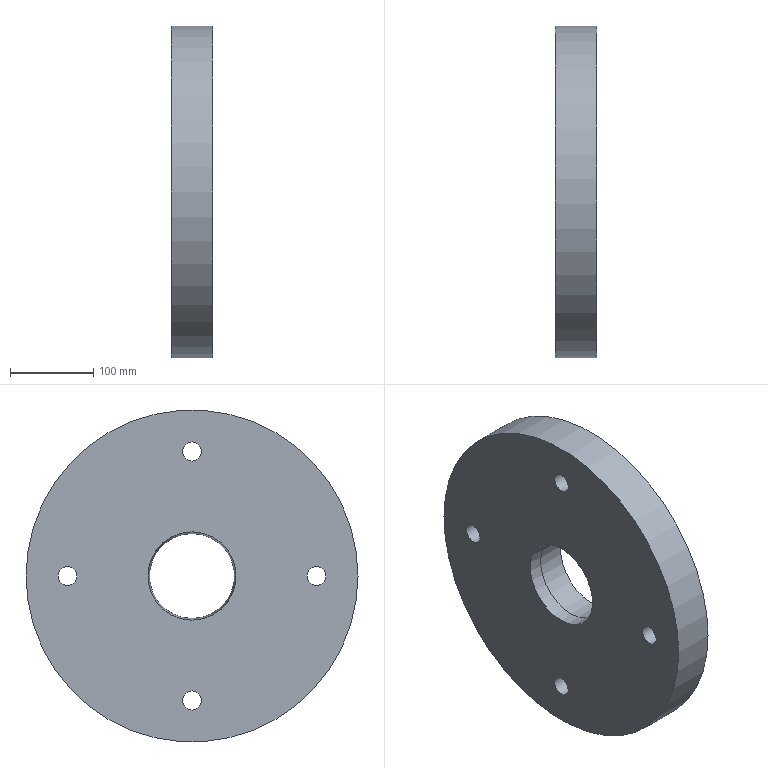Component | NX | ADAPTER_PLATE | 1 solid | 9 faces | box 50 x 400 x 400 mm | volume 5783300 mm3 | cylinder 6 | plane 2 | cone 1 | commonest cylinder face diameters 23 x4 400 x1 102.376 x1
STEP:
#1=CARTESIAN_POINT('',(0.,0.,0.));
#2=DIRECTION('',(0.,0.,1.));
#3=DIRECTION('',(1.,0.,0.));
#4=AXIS2_PLACEMENT_3D('',#1,#2,#3);
#5=CARTESIAN_POINT('',(0.,200.,-0.));
#6=VERTEX_POINT('',#5);
#7=CARTESIAN_POINT('',(0.,0.,0.));
#8=DIRECTION('',(1.,0.,0.));
#9=DIRECTION('',(0.,1.,-0.));
#10=AXIS2_PLACEMENT_3D('',#7,#8,#9);
#11=CIRCLE('',#10,200.);
#12=CARTESIAN_POINT('',(0.,0.,0.));
#13=DIRECTION('',(-1.,0.,0.));
#14=DIRECTION('',(0.,0.,1.));
#15=AXIS2_PLACEMENT_3D('',#12,#13,#14);
#16=CYLINDRICAL_SURFACE('',#15,200.);
#17=CARTESIAN_POINT('',(7.854,0.));
#18=DIRECTION('',(-1.,0.));
#19=VECTOR('',#18,1.);
#20=LINE('',#17,#19);
#21=(GEOMETRIC_REPRESENTATION_CONTEXT(2)PARAMETRIC_REPRESENTATION_CONTEXT()REPRESENTATION_CONTEXT('',''));
#22=DEFINITIONAL_REPRESENTATION('',(#20),#21);
#23=PCURVE('',#16,#22);
#24=CARTESIAN_POINT('',(0.,0.,0.));
#25=DIRECTION('',(1.,0.,0.));
#26=DIRECTION('',(0.,0.,-1.));
#27=AXIS2_PLACEMENT_3D('',#24,#25,#26);
#28=PLANE('',#27);
#29=CARTESIAN_POINT('',(0.,0.));
#30=DIRECTION('',(0.,1.));
#31=AXIS2_PLACEMENT_2D('',#29,#30);
#32=CIRCLE('',#31,200.);
#33=(GEOMETRIC_REPRESENTATION_CONTEXT(2)PARAMETRIC_REPRESENTATION_CONTEXT()REPRESENTATION_CONTEXT('',''));
#34=DEFINITIONAL_REPRESENTATION('',(#32),#33);
#35=PCURVE('',#28,#34);
#36=SURFACE_CURVE('',#11,(#23,#35),.PCURVE_S1.);
#37=EDGE_CURVE('',#6,#6,#36,.T.);
#38=ORIENTED_EDGE('',*,*,#37,.F.);
#39=CARTESIAN_POINT('',(-50.,200.,-0.));
#40=VERTEX_POINT('',#39);
#41=CARTESIAN_POINT('',(0.,200.,0.));
#42=CARTESIAN_POINT('',(-50.,200.,0.));
#43=B_SPLINE_CURVE_WITH_KNOTS('',1,(#41,#42),.UNSPECIFIED.,.F.,.F.,(2,2),(0.,50.),.PIECEWISE_BEZIER_KNOTS.);
#44=CARTESIAN_POINT('',(7.854,0.));
#45=DIRECTION('',(0.,1.));
#46=VECTOR('',#45,1.);
#47=LINE('',#44,#46);
#48=(GEOMETRIC_REPRESENTATION_CONTEXT(2)PARAMETRIC_REPRESENTATION_CONTEXT()REPRESENTATION_CONTEXT('',''));
#49=DEFINITIONAL_REPRESENTATION('',(#47),#48);
#50=PCURVE('',#16,#49);
#51=CARTESIAN_POINT('',(1.571,0.));
#52=DIRECTION('',(0.,1.));
#53=VECTOR('',#52,1.);
#54=LINE('',#51,#53);
#55=(GEOMETRIC_REPRESENTATION_CONTEXT(2)PARAMETRIC_REPRESENTATION_CONTEXT()REPRESENTATION_CONTEXT('',''));
#56=DEFINITIONAL_REPRESENTATION('',(#54),#55);
#57=PCURVE('',#16,#56);
#58=SEAM_CURVE('',#43,(#50,#57),.PCURVE_S1.);
#59=EDGE_CURVE('',#6,#40,#58,.T.);
#60=ORIENTED_EDGE('',*,*,#59,.T.);
#61=CARTESIAN_POINT('',(-50.,0.,0.));
#62=DIRECTION('',(1.,0.,0.));
#63=DIRECTION('',(0.,1.,-0.));
#64=AXIS2_PLACEMENT_3D('',#61,#62,#63);
#65=CIRCLE('',#64,200.);
#66=CARTESIAN_POINT('',(7.854,50.));
#67=DIRECTION('',(-1.,0.));
#68=VECTOR('',#67,1.);
#69=LINE('',#66,#68);
#70=(GEOMETRIC_REPRESENTATION_CONTEXT(2)PARAMETRIC_REPRESENTATION_CONTEXT()REPRESENTATION_CONTEXT('',''));
#71=DEFINITIONAL_REPRESENTATION('',(#69),#70);
#72=PCURVE('',#16,#71);
#73=CARTESIAN_POINT('',(-50.,0.,0.));
#74=DIRECTION('',(1.,0.,0.));
#75=DIRECTION('',(0.,0.,-1.));
#76=AXIS2_PLACEMENT_3D('',#73,#74,#75);
#77=PLANE('',#76);
#78=CARTESIAN_POINT('',(0.,0.));
#79=DIRECTION('',(0.,1.));
#80=AXIS2_PLACEMENT_2D('',#78,#79);
#81=CIRCLE('',#80,200.);
#82=(GEOMETRIC_REPRESENTATION_CONTEXT(2)PARAMETRIC_REPRESENTATION_CONTEXT()REPRESENTATION_CONTEXT('',''));
#83=DEFINITIONAL_REPRESENTATION('',(#81),#82);
#84=PCURVE('',#77,#83);
#85=SURFACE_CURVE('',#65,(#72,#84),.PCURVE_S1.);
#86=EDGE_CURVE('',#40,#40,#85,.T.);
#87=ORIENTED_EDGE('',*,*,#86,.T.);
#88=ORIENTED_EDGE('',*,*,#59,.F.);
#89=EDGE_LOOP('',(#38,#60,#87,#88));
#90=FACE_BOUND('',#89,.T.);
#91=ADVANCED_FACE('',(#90),#16,.T.);
#92=CARTESIAN_POINT('',(0.,150.,-11.5));
#93=VERTEX_POINT('',#92);
#94=CARTESIAN_POINT('',(0.,150.,0.));
#95=DIRECTION('',(1.,0.,0.));
#96=DIRECTION('',(0.,0.,-1.));
#97=AXIS2_PLACEMENT_3D('',#94,#95,#96);
#98=CIRCLE('',#97,11.5);
#99=CARTESIAN_POINT('',(0.,150.));
#100=DIRECTION('',(1.,0.));
#101=AXIS2_PLACEMENT_2D('',#99,#100);
#102=CIRCLE('',#101,11.5);
#103=(GEOMETRIC_REPRESENTATION_CONTEXT(2)PARAMETRIC_REPRESENTATION_CONTEXT()REPRESENTATION_CONTEXT('',''));
#104=DEFINITIONAL_REPRESENTATION('',(#102),#103);
#105=PCURVE('',#28,#104);
#106=CARTESIAN_POINT('',(-50.,150.,0.));
#107=DIRECTION('',(1.,0.,0.));
#108=DIRECTION('',(0.,0.,-1.));
#109=AXIS2_PLACEMENT_3D('',#106,#107,#108);
#110=CYLINDRICAL_SURFACE('',#109,11.5);
#111=CARTESIAN_POINT('',(0.,50.));
#112=DIRECTION('',(1.,0.));
#113=VECTOR('',#112,1.);
#114=LINE('',#111,#113);
#115=(GEOMETRIC_REPRESENTATION_CONTEXT(2)PARAMETRIC_REPRESENTATION_CONTEXT()REPRESENTATION_CONTEXT('',''));
#116=DEFINITIONAL_REPRESENTATION('',(#114),#115);
#117=PCURVE('',#110,#116);
#118=SURFACE_CURVE('',#98,(#105,#117),.PCURVE_S1.);
#119=EDGE_CURVE('',#93,#93,#118,.T.);
#120=ORIENTED_EDGE('',*,*,#119,.F.);
#121=EDGE_LOOP('',(#120));
#122=FACE_BOUND('',#121,.T.);
#123=CARTESIAN_POINT('',(0.,0.,138.5));
#124=VERTEX_POINT('',#123);
#125=CARTESIAN_POINT('',(0.,0.,150.));
#126=DIRECTION('',(1.,0.,0.));
#127=DIRECTION('',(0.,0.,-1.));
#128=AXIS2_PLACEMENT_3D('',#125,#126,#127);
#129=CIRCLE('',#128,11.5);
#130=CARTESIAN_POINT('',(-150.,0.));
#131=DIRECTION('',(1.,0.));
#132=AXIS2_PLACEMENT_2D('',#130,#131);
#133=CIRCLE('',#132,11.5);
#134=(GEOMETRIC_REPRESENTATION_CONTEXT(2)PARAMETRIC_REPRESENTATION_CONTEXT()REPRESENTATION_CONTEXT('',''));
#135=DEFINITIONAL_REPRESENTATION('',(#133),#134);
#136=PCURVE('',#28,#135);
#137=CARTESIAN_POINT('',(-50.,0.,150.));
#138=DIRECTION('',(1.,0.,0.));
#139=DIRECTION('',(0.,0.,-1.));
#140=AXIS2_PLACEMENT_3D('',#137,#138,#139);
#141=CYLINDRICAL_SURFACE('',#140,11.5);
#142=CARTESIAN_POINT('',(0.,50.));
#143=DIRECTION('',(1.,0.));
#144=VECTOR('',#143,1.);
#145=LINE('',#142,#144);
#146=(GEOMETRIC_REPRESENTATION_CONTEXT(2)PARAMETRIC_REPRESENTATION_CONTEXT()REPRESENTATION_CONTEXT('',''));
#147=DEFINITIONAL_REPRESENTATION('',(#145),#146);
#148=PCURVE('',#141,#147);
#149=SURFACE_CURVE('',#129,(#136,#148),.PCURVE_S1.);
#150=EDGE_CURVE('',#124,#124,#149,.T.);
#151=ORIENTED_EDGE('',*,*,#150,.F.);
#152=EDGE_LOOP('',(#151));
#153=FACE_BOUND('',#152,.T.);
#154=CARTESIAN_POINT('',(0.,0.,-161.5));
#155=VERTEX_POINT('',#154);
#156=CARTESIAN_POINT('',(0.,0.,-150.));
#157=DIRECTION('',(1.,0.,0.));
#158=DIRECTION('',(0.,0.,-1.));
#159=AXIS2_PLACEMENT_3D('',#156,#157,#158);
#160=CIRCLE('',#159,11.5);
#161=CARTESIAN_POINT('',(150.,0.));
#162=DIRECTION('',(1.,0.));
#163=AXIS2_PLACEMENT_2D('',#161,#162);
#164=CIRCLE('',#163,11.5);
#165=(GEOMETRIC_REPRESENTATION_CONTEXT(2)PARAMETRIC_REPRESENTATION_CONTEXT()REPRESENTATION_CONTEXT('',''));
#166=DEFINITIONAL_REPRESENTATION('',(#164),#165);
#167=PCURVE('',#28,#166);
#168=CARTESIAN_POINT('',(-50.,0.,-150.));
#169=DIRECTION('',(1.,0.,0.));
#170=DIRECTION('',(0.,0.,-1.));
#171=AXIS2_PLACEMENT_3D('',#168,#169,#170);
#172=CYLINDRICAL_SURFACE('',#171,11.5);
#173=CARTESIAN_POINT('',(0.,50.));
#174=DIRECTION('',(1.,0.));
#175=VECTOR('',#174,1.);
#176=LINE('',#173,#175);
#177=(GEOMETRIC_REPRESENTATION_CONTEXT(2)PARAMETRIC_REPRESENTATION_CONTEXT()REPRESENTATION_CONTEXT('',''));
#178=DEFINITIONAL_REPRESENTATION('',(#176),#177);
#179=PCURVE('',#172,#178);
#180=SURFACE_CURVE('',#160,(#167,#179),.PCURVE_S1.);
#181=EDGE_CURVE('',#155,#155,#180,.T.);
#182=ORIENTED_EDGE('',*,*,#181,.F.);
#183=EDGE_LOOP('',(#182));
#184=FACE_BOUND('',#183,.T.);
#185=CARTESIAN_POINT('',(0.,-150.,-11.5));
#186=VERTEX_POINT('',#185);
#187=CARTESIAN_POINT('',(0.,-150.,0.));
#188=DIRECTION('',(1.,0.,0.));
#189=DIRECTION('',(0.,0.,-1.));
#190=AXIS2_PLACEMENT_3D('',#187,#188,#189);
#191=CIRCLE('',#190,11.5);
#192=CARTESIAN_POINT('',(0.,-150.));
#193=DIRECTION('',(1.,0.));
#194=AXIS2_PLACEMENT_2D('',#192,#193);
#195=CIRCLE('',#194,11.5);
#196=(GEOMETRIC_REPRESENTATION_CONTEXT(2)PARAMETRIC_REPRESENTATION_CONTEXT()REPRESENTATION_CONTEXT('',''));
#197=DEFINITIONAL_REPRESENTATION('',(#195),#196);
#198=PCURVE('',#28,#197);
#199=CARTESIAN_POINT('',(-50.,-150.,0.));
#200=DIRECTION('',(1.,0.,0.));
#201=DIRECTION('',(0.,0.,-1.));
#202=AXIS2_PLACEMENT_3D('',#199,#200,#201);
#203=CYLINDRICAL_SURFACE('',#202,11.5);
#204=CARTESIAN_POINT('',(0.,50.));
#205=DIRECTION('',(1.,0.));
#206=VECTOR('',#205,1.);
#207=LINE('',#204,#206);
#208=(GEOMETRIC_REPRESENTATION_CONTEXT(2)PARAMETRIC_REPRESENTATION_CONTEXT()REPRESENTATION_CONTEXT('',''));
#209=DEFINITIONAL_REPRESENTATION('',(#207),#208);
#210=PCURVE('',#203,#209);
#211=SURFACE_CURVE('',#191,(#198,#210),.PCURVE_S1.);
#212=EDGE_CURVE('',#186,#186,#211,.T.);
#213=ORIENTED_EDGE('',*,*,#212,.F.);
#214=EDGE_LOOP('',(#213));
#215=FACE_BOUND('',#214,.T.);
#216=CARTESIAN_POINT('',(0.,0.,-51.188));
#217=VERTEX_POINT('',#216);
#218=CARTESIAN_POINT('',(0.,-0.,51.188));
#219=VERTEX_POINT('',#218);
#220=CARTESIAN_POINT('',(0.,0.,0.));
#221=DIRECTION('',(-1.,0.,0.));
#222=DIRECTION('',(0.,0.,-1.));
#223=AXIS2_PLACEMENT_3D('',#220,#221,#222);
#224=CIRCLE('',#223,51.188);
#225=CARTESIAN_POINT('',(51.188,0.));
#226=CARTESIAN_POINT('',(51.188,-88.66));
#227=CARTESIAN_POINT('',(-25.594,-44.33));
#228=CARTESIAN_POINT('',(-102.376,-0.));
#229=CARTESIAN_POINT('',(-25.594,44.33));
#230=CARTESIAN_POINT('',(51.188,88.66));
#231=CARTESIAN_POINT('',(51.188,0.));
#232=(BOUNDED_CURVE()B_SPLINE_CURVE(2,(#225,#226,#227,#228,#229,#230,#231),.UNSPECIFIED.,.T.,.F.)B_SPLINE_CURVE_WITH_KNOTS((1,2,2,2,2,1),(-2.094,0.,2.094,4.189,6.283,8.378),.UNSPECIFIED.)CURVE()GEOMETRIC_REPRESENTATION_ITEM()RATIONAL_B_SPLINE_CURVE((1.,0.5,1.,0.5,1.,0.5,1.))REPRESENTATION_ITEM(''));
#233=(GEOMETRIC_REPRESENTATION_CONTEXT(2)PARAMETRIC_REPRESENTATION_CONTEXT()REPRESENTATION_CONTEXT('',''));
#234=DEFINITIONAL_REPRESENTATION('',(#232),#233);
#235=PCURVE('',#28,#234);
#236=CARTESIAN_POINT('',(0.,0.,0.));
#237=DIRECTION('',(-1.,0.,0.));
#238=DIRECTION('',(0.,0.,1.));
#239=AXIS2_PLACEMENT_3D('',#236,#237,#238);
#240=CYLINDRICAL_SURFACE('',#239,51.188);
#241=CARTESIAN_POINT('',(3.142,0.));
#242=DIRECTION('',(1.,0.));
#243=VECTOR('',#242,1.);
#244=LINE('',#241,#243);
#245=(GEOMETRIC_REPRESENTATION_CONTEXT(2)PARAMETRIC_REPRESENTATION_CONTEXT()REPRESENTATION_CONTEXT('',''));
#246=DEFINITIONAL_REPRESENTATION('',(#244),#245);
#247=PCURVE('',#240,#246);
#248=SURFACE_CURVE('',#224,(#235,#247),.PCURVE_S1.);
#249=EDGE_CURVE('',#217,#219,#248,.T.);
#250=ORIENTED_EDGE('',*,*,#249,.T.);
#251=CARTESIAN_POINT('',(0.,0.,0.));
#252=DIRECTION('',(-1.,0.,0.));
#253=DIRECTION('',(0.,0.,-1.));
#254=AXIS2_PLACEMENT_3D('',#251,#252,#253);
#255=CIRCLE('',#254,51.188);
#256=CARTESIAN_POINT('',(51.188,0.));
#257=CARTESIAN_POINT('',(51.188,-88.66));
#258=CARTESIAN_POINT('',(-25.594,-44.33));
#259=CARTESIAN_POINT('',(-102.376,-0.));
#260=CARTESIAN_POINT('',(-25.594,44.33));
#261=CARTESIAN_POINT('',(51.188,88.66));
#262=CARTESIAN_POINT('',(51.188,0.));
#263=(BOUNDED_CURVE()B_SPLINE_CURVE(2,(#256,#257,#258,#259,#260,#261,#262),.UNSPECIFIED.,.T.,.F.)B_SPLINE_CURVE_WITH_KNOTS((1,2,2,2,2,1),(-2.094,0.,2.094,4.189,6.283,8.378),.UNSPECIFIED.)CURVE()GEOMETRIC_REPRESENTATION_ITEM()RATIONAL_B_SPLINE_CURVE((1.,0.5,1.,0.5,1.,0.5,1.))REPRESENTATION_ITEM(''));
#264=(GEOMETRIC_REPRESENTATION_CONTEXT(2)PARAMETRIC_REPRESENTATION_CONTEXT()REPRESENTATION_CONTEXT('',''));
#265=DEFINITIONAL_REPRESENTATION('',(#263),#264);
#266=PCURVE('',#28,#265);
#267=CARTESIAN_POINT('',(-3.142,0.));
#268=DIRECTION('',(1.,0.));
#269=VECTOR('',#268,1.);
#270=LINE('',#267,#269);
#271=(GEOMETRIC_REPRESENTATION_CONTEXT(2)PARAMETRIC_REPRESENTATION_CONTEXT()REPRESENTATION_CONTEXT('',''));
#272=DEFINITIONAL_REPRESENTATION('',(#270),#271);
#273=PCURVE('',#240,#272);
#274=SURFACE_CURVE('',#255,(#266,#273),.PCURVE_S1.);
#275=EDGE_CURVE('',#219,#217,#274,.T.);
#276=ORIENTED_EDGE('',*,*,#275,.T.);
#277=EDGE_LOOP('',(#250,#276));
#278=FACE_BOUND('',#277,.T.);
#279=ORIENTED_EDGE('',*,*,#37,.T.);
#280=EDGE_LOOP('',(#279));
#281=FACE_BOUND('',#280,.T.);
#282=ADVANCED_FACE('',(#122,#153,#184,#215,#278,#281),#28,.T.);
#283=CARTESIAN_POINT('',(-50.,150.,-11.5));
#284=VERTEX_POINT('',#283);
#285=CARTESIAN_POINT('',(-50.,150.,0.));
#286=DIRECTION('',(1.,0.,0.));
#287=DIRECTION('',(0.,0.,-1.));
#288=AXIS2_PLACEMENT_3D('',#285,#286,#287);
#289=CIRCLE('',#288,11.5);
#290=CARTESIAN_POINT('',(0.,150.));
#291=DIRECTION('',(1.,0.));
#292=AXIS2_PLACEMENT_2D('',#290,#291);
#293=CIRCLE('',#292,11.5);
#294=(GEOMETRIC_REPRESENTATION_CONTEXT(2)PARAMETRIC_REPRESENTATION_CONTEXT()REPRESENTATION_CONTEXT('',''));
#295=DEFINITIONAL_REPRESENTATION('',(#293),#294);
#296=PCURVE('',#77,#295);
#297=CARTESIAN_POINT('',(0.,0.));
#298=DIRECTION('',(1.,0.));
#299=VECTOR('',#298,1.);
#300=LINE('',#297,#299);
#301=(GEOMETRIC_REPRESENTATION_CONTEXT(2)PARAMETRIC_REPRESENTATION_CONTEXT()REPRESENTATION_CONTEXT('',''));
#302=DEFINITIONAL_REPRESENTATION('',(#300),#301);
#303=PCURVE('',#110,#302);
#304=SURFACE_CURVE('',#289,(#296,#303),.PCURVE_S1.);
#305=EDGE_CURVE('',#284,#284,#304,.T.);
#306=ORIENTED_EDGE('',*,*,#305,.T.);
#307=EDGE_LOOP('',(#306));
#308=FACE_BOUND('',#307,.T.);
#309=CARTESIAN_POINT('',(-50.,0.,138.5));
#310=VERTEX_POINT('',#309);
#311=CARTESIAN_POINT('',(-50.,0.,150.));
#312=DIRECTION('',(1.,0.,0.));
#313=DIRECTION('',(0.,0.,-1.));
#314=AXIS2_PLACEMENT_3D('',#311,#312,#313);
#315=CIRCLE('',#314,11.5);
#316=CARTESIAN_POINT('',(-150.,0.));
#317=DIRECTION('',(1.,0.));
#318=AXIS2_PLACEMENT_2D('',#316,#317);
#319=CIRCLE('',#318,11.5);
#320=(GEOMETRIC_REPRESENTATION_CONTEXT(2)PARAMETRIC_REPRESENTATION_CONTEXT()REPRESENTATION_CONTEXT('',''));
#321=DEFINITIONAL_REPRESENTATION('',(#319),#320);
#322=PCURVE('',#77,#321);
#323=CARTESIAN_POINT('',(0.,0.));
#324=DIRECTION('',(1.,0.));
#325=VECTOR('',#324,1.);
#326=LINE('',#323,#325);
#327=(GEOMETRIC_REPRESENTATION_CONTEXT(2)PARAMETRIC_REPRESENTATION_CONTEXT()REPRESENTATION_CONTEXT('',''));
#328=DEFINITIONAL_REPRESENTATION('',(#326),#327);
#329=PCURVE('',#141,#328);
#330=SURFACE_CURVE('',#315,(#322,#329),.PCURVE_S1.);
#331=EDGE_CURVE('',#310,#310,#330,.T.);
#332=ORIENTED_EDGE('',*,*,#331,.T.);
#333=EDGE_LOOP('',(#332));
#334=FACE_BOUND('',#333,.T.);
#335=CARTESIAN_POINT('',(-50.,0.,-161.5));
#336=VERTEX_POINT('',#335);
#337=CARTESIAN_POINT('',(-50.,0.,-150.));
#338=DIRECTION('',(1.,0.,0.));
#339=DIRECTION('',(0.,0.,-1.));
#340=AXIS2_PLACEMENT_3D('',#337,#338,#339);
#341=CIRCLE('',#340,11.5);
#342=CARTESIAN_POINT('',(150.,0.));
#343=DIRECTION('',(1.,0.));
#344=AXIS2_PLACEMENT_2D('',#342,#343);
#345=CIRCLE('',#344,11.5);
#346=(GEOMETRIC_REPRESENTATION_CONTEXT(2)PARAMETRIC_REPRESENTATION_CONTEXT()REPRESENTATION_CONTEXT('',''));
#347=DEFINITIONAL_REPRESENTATION('',(#345),#346);
#348=PCURVE('',#77,#347);
#349=CARTESIAN_POINT('',(0.,0.));
#350=DIRECTION('',(1.,0.));
#351=VECTOR('',#350,1.);
#352=LINE('',#349,#351);
#353=(GEOMETRIC_REPRESENTATION_CONTEXT(2)PARAMETRIC_REPRESENTATION_CONTEXT()REPRESENTATION_CONTEXT('',''));
#354=DEFINITIONAL_REPRESENTATION('',(#352),#353);
#355=PCURVE('',#172,#354);
#356=SURFACE_CURVE('',#341,(#348,#355),.PCURVE_S1.);
#357=EDGE_CURVE('',#336,#336,#356,.T.);
#358=ORIENTED_EDGE('',*,*,#357,.T.);
#359=EDGE_LOOP('',(#358));
#360=FACE_BOUND('',#359,.T.);
#361=CARTESIAN_POINT('',(-50.,-150.,-11.5));
#362=VERTEX_POINT('',#361);
#363=CARTESIAN_POINT('',(-50.,-150.,0.));
#364=DIRECTION('',(1.,0.,0.));
#365=DIRECTION('',(0.,0.,-1.));
#366=AXIS2_PLACEMENT_3D('',#363,#364,#365);
#367=CIRCLE('',#366,11.5);
#368=CARTESIAN_POINT('',(0.,-150.));
#369=DIRECTION('',(1.,0.));
#370=AXIS2_PLACEMENT_2D('',#368,#369);
#371=CIRCLE('',#370,11.5);
#372=(GEOMETRIC_REPRESENTATION_CONTEXT(2)PARAMETRIC_REPRESENTATION_CONTEXT()REPRESENTATION_CONTEXT('',''));
#373=DEFINITIONAL_REPRESENTATION('',(#371),#372);
#374=PCURVE('',#77,#373);
#375=CARTESIAN_POINT('',(0.,0.));
#376=DIRECTION('',(1.,0.));
#377=VECTOR('',#376,1.);
#378=LINE('',#375,#377);
#379=(GEOMETRIC_REPRESENTATION_CONTEXT(2)PARAMETRIC_REPRESENTATION_CONTEXT()REPRESENTATION_CONTEXT('',''));
#380=DEFINITIONAL_REPRESENTATION('',(#378),#379);
#381=PCURVE('',#203,#380);
#382=SURFACE_CURVE('',#367,(#374,#381),.PCURVE_S1.);
#383=EDGE_CURVE('',#362,#362,#382,.T.);
#384=ORIENTED_EDGE('',*,*,#383,.T.);
#385=EDGE_LOOP('',(#384));
#386=FACE_BOUND('',#385,.T.);
#387=CARTESIAN_POINT('',(-50.,0.,53.187));
#388=VERTEX_POINT('',#387);
#389=CARTESIAN_POINT('',(-50.,0.,0.));
#390=DIRECTION('',(-1.,0.,0.));
#391=DIRECTION('',(0.,0.,1.));
#392=AXIS2_PLACEMENT_3D('',#389,#390,#391);
#393=CIRCLE('',#392,53.187);
#394=CARTESIAN_POINT('',(-53.187,0.));
#395=CARTESIAN_POINT('',(-53.187,92.122));
#396=CARTESIAN_POINT('',(26.593,46.061));
#397=CARTESIAN_POINT('',(106.373,0.));
#398=CARTESIAN_POINT('',(26.593,-46.061));
#399=CARTESIAN_POINT('',(-53.187,-92.122));
#400=CARTESIAN_POINT('',(-53.187,0.));
#401=(BOUNDED_CURVE()B_SPLINE_CURVE(2,(#394,#395,#396,#397,#398,#399,#400),.UNSPECIFIED.,.T.,.F.)B_SPLINE_CURVE_WITH_KNOTS((1,2,2,2,2,1),(-2.094,0.,2.094,4.189,6.283,8.378),.UNSPECIFIED.)CURVE()GEOMETRIC_REPRESENTATION_ITEM()RATIONAL_B_SPLINE_CURVE((1.,0.5,1.,0.5,1.,0.5,1.))REPRESENTATION_ITEM(''));
#402=(GEOMETRIC_REPRESENTATION_CONTEXT(2)PARAMETRIC_REPRESENTATION_CONTEXT()REPRESENTATION_CONTEXT('',''));
#403=DEFINITIONAL_REPRESENTATION('',(#401),#402);
#404=PCURVE('',#77,#403);
#405=CARTESIAN_POINT('',(-34.,0.,0.));
#406=DIRECTION('',(-1.,0.,0.));
#407=DIRECTION('',(0.,0.,1.));
#408=AXIS2_PLACEMENT_3D('',#405,#406,#407);
#409=CONICAL_SURFACE('',#408,51.188,0.1243);
#410=CARTESIAN_POINT('',(0.,16.));
#411=DIRECTION('',(1.,0.));
#412=VECTOR('',#411,1.);
#413=LINE('',#410,#412);
#414=(GEOMETRIC_REPRESENTATION_CONTEXT(2)PARAMETRIC_REPRESENTATION_CONTEXT()REPRESENTATION_CONTEXT('',''));
#415=DEFINITIONAL_REPRESENTATION('',(#413),#414);
#416=PCURVE('',#409,#415);
#417=SURFACE_CURVE('',#393,(#404,#416),.PCURVE_S1.);
#418=EDGE_CURVE('',#388,#388,#417,.T.);
#419=ORIENTED_EDGE('',*,*,#418,.F.);
#420=EDGE_LOOP('',(#419));
#421=FACE_BOUND('',#420,.T.);
#422=ORIENTED_EDGE('',*,*,#86,.F.);
#423=EDGE_LOOP('',(#422));
#424=FACE_BOUND('',#423,.T.);
#425=ADVANCED_FACE('',(#308,#334,#360,#386,#421,#424),#77,.F.);
#426=ORIENTED_EDGE('',*,*,#418,.F.);
#427=CARTESIAN_POINT('',(-34.,0.,51.188));
#428=VERTEX_POINT('',#427);
#429=CARTESIAN_POINT('',(-34.,-0.,51.188));
#430=CARTESIAN_POINT('',(-50.,-0.,53.186));
#431=B_SPLINE_CURVE_WITH_KNOTS('',1,(#429,#430),.UNSPECIFIED.,.F.,.F.,(2,2),(0.,16.124),.PIECEWISE_BEZIER_KNOTS.);
#432=CARTESIAN_POINT('',(0.,0.));
#433=DIRECTION('',(0.,1.));
#434=VECTOR('',#433,1.);
#435=LINE('',#432,#434);
#436=(GEOMETRIC_REPRESENTATION_CONTEXT(2)PARAMETRIC_REPRESENTATION_CONTEXT()REPRESENTATION_CONTEXT('',''));
#437=DEFINITIONAL_REPRESENTATION('',(#435),#436);
#438=PCURVE('',#409,#437);
#439=CARTESIAN_POINT('',(6.283,0.));
#440=DIRECTION('',(0.,1.));
#441=VECTOR('',#440,1.);
#442=LINE('',#439,#441);
#443=(GEOMETRIC_REPRESENTATION_CONTEXT(2)PARAMETRIC_REPRESENTATION_CONTEXT()REPRESENTATION_CONTEXT('',''));
#444=DEFINITIONAL_REPRESENTATION('',(#442),#443);
#445=PCURVE('',#409,#444);
#446=SEAM_CURVE('',#431,(#438,#445),.PCURVE_S1.);
#447=EDGE_CURVE('',#428,#388,#446,.T.);
#448=ORIENTED_EDGE('',*,*,#447,.F.);
#449=CARTESIAN_POINT('',(-34.,0.,0.));
#450=DIRECTION('',(1.,0.,0.));
#451=DIRECTION('',(0.,0.,1.));
#452=AXIS2_PLACEMENT_3D('',#449,#450,#451);
#453=CIRCLE('',#452,51.188);
#454=CARTESIAN_POINT('',(6.283,0.));
#455=DIRECTION('',(-1.,0.));
#456=VECTOR('',#455,1.);
#457=LINE('',#454,#456);
#458=(GEOMETRIC_REPRESENTATION_CONTEXT(2)PARAMETRIC_REPRESENTATION_CONTEXT()REPRESENTATION_CONTEXT('',''));
#459=DEFINITIONAL_REPRESENTATION('',(#457),#458);
#460=PCURVE('',#409,#459);
#461=CARTESIAN_POINT('',(6.283,34.));
#462=DIRECTION('',(-1.,0.));
#463=VECTOR('',#462,1.);
#464=LINE('',#461,#463);
#465=(GEOMETRIC_REPRESENTATION_CONTEXT(2)PARAMETRIC_REPRESENTATION_CONTEXT()REPRESENTATION_CONTEXT('',''));
#466=DEFINITIONAL_REPRESENTATION('',(#464),#465);
#467=PCURVE('',#240,#466);
#468=SURFACE_CURVE('',#453,(#460,#467),.PCURVE_S1.);
#469=EDGE_CURVE('',#428,#428,#468,.T.);
#470=ORIENTED_EDGE('',*,*,#469,.F.);
#471=ORIENTED_EDGE('',*,*,#447,.T.);
#472=EDGE_LOOP('',(#426,#448,#470,#471));
#473=FACE_BOUND('',#472,.F.);
#474=ADVANCED_FACE('',(#473),#409,.F.);
#475=ORIENTED_EDGE('',*,*,#249,.T.);
#476=CARTESIAN_POINT('',(0.,0.,51.188));
#477=CARTESIAN_POINT('',(-34.,0.,51.188));
#478=B_SPLINE_CURVE_WITH_KNOTS('',1,(#476,#477),.UNSPECIFIED.,.F.,.F.,(2,2),(0.,34.),.PIECEWISE_BEZIER_KNOTS.);
#479=CARTESIAN_POINT('',(6.283,0.));
#480=DIRECTION('',(0.,1.));
#481=VECTOR('',#480,1.);
#482=LINE('',#479,#481);
#483=(GEOMETRIC_REPRESENTATION_CONTEXT(2)PARAMETRIC_REPRESENTATION_CONTEXT()REPRESENTATION_CONTEXT('',''));
#484=DEFINITIONAL_REPRESENTATION('',(#482),#483);
#485=PCURVE('',#240,#484);
#486=CARTESIAN_POINT('',(0.,0.));
#487=DIRECTION('',(0.,1.));
#488=VECTOR('',#487,1.);
#489=LINE('',#486,#488);
#490=(GEOMETRIC_REPRESENTATION_CONTEXT(2)PARAMETRIC_REPRESENTATION_CONTEXT()REPRESENTATION_CONTEXT('',''));
#491=DEFINITIONAL_REPRESENTATION('',(#489),#490);
#492=PCURVE('',#240,#491);
#493=SEAM_CURVE('',#478,(#485,#492),.PCURVE_S1.);
#494=EDGE_CURVE('',#219,#428,#493,.T.);
#495=ORIENTED_EDGE('',*,*,#494,.T.);
#496=ORIENTED_EDGE('',*,*,#469,.T.);
#497=ORIENTED_EDGE('',*,*,#494,.F.);
#498=ORIENTED_EDGE('',*,*,#275,.T.);
#499=EDGE_LOOP('',(#475,#495,#496,#497,#498));
#500=FACE_BOUND('',#499,.F.);
#501=ADVANCED_FACE('',(#500),#240,.F.);
#502=ORIENTED_EDGE('',*,*,#212,.F.);
#503=CARTESIAN_POINT('',(-50.,-150.,-11.5));
#504=CARTESIAN_POINT('',(0.,-150.,-11.5));
#505=B_SPLINE_CURVE_WITH_KNOTS('',1,(#503,#504),.UNSPECIFIED.,.F.,.F.,(2,2),(0.,50.),.PIECEWISE_BEZIER_KNOTS.);
#506=CARTESIAN_POINT('',(0.,0.));
#507=DIRECTION('',(0.,1.));
#508=VECTOR('',#507,1.);
#509=LINE('',#506,#508);
#510=(GEOMETRIC_REPRESENTATION_CONTEXT(2)PARAMETRIC_REPRESENTATION_CONTEXT()REPRESENTATION_CONTEXT('',''));
#511=DEFINITIONAL_REPRESENTATION('',(#509),#510);
#512=PCURVE('',#203,#511);
#513=CARTESIAN_POINT('',(6.283,0.));
#514=DIRECTION('',(0.,1.));
#515=VECTOR('',#514,1.);
#516=LINE('',#513,#515);
#517=(GEOMETRIC_REPRESENTATION_CONTEXT(2)PARAMETRIC_REPRESENTATION_CONTEXT()REPRESENTATION_CONTEXT('',''));
#518=DEFINITIONAL_REPRESENTATION('',(#516),#517);
#519=PCURVE('',#203,#518);
#520=SEAM_CURVE('',#505,(#512,#519),.PCURVE_S1.);
#521=EDGE_CURVE('',#362,#186,#520,.T.);
#522=ORIENTED_EDGE('',*,*,#521,.F.);
#523=ORIENTED_EDGE('',*,*,#383,.T.);
#524=ORIENTED_EDGE('',*,*,#521,.T.);
#525=EDGE_LOOP('',(#502,#522,#523,#524));
#526=FACE_BOUND('',#525,.F.);
#527=ADVANCED_FACE('',(#526),#203,.F.);
#528=ORIENTED_EDGE('',*,*,#181,.F.);
#529=CARTESIAN_POINT('',(-50.,-0.,-161.5));
#530=CARTESIAN_POINT('',(0.,-0.,-161.5));
#531=B_SPLINE_CURVE_WITH_KNOTS('',1,(#529,#530),.UNSPECIFIED.,.F.,.F.,(2,2),(0.,50.),.PIECEWISE_BEZIER_KNOTS.);
#532=CARTESIAN_POINT('',(0.,0.));
#533=DIRECTION('',(0.,1.));
#534=VECTOR('',#533,1.);
#535=LINE('',#532,#534);
#536=(GEOMETRIC_REPRESENTATION_CONTEXT(2)PARAMETRIC_REPRESENTATION_CONTEXT()REPRESENTATION_CONTEXT('',''));
#537=DEFINITIONAL_REPRESENTATION('',(#535),#536);
#538=PCURVE('',#172,#537);
#539=CARTESIAN_POINT('',(6.283,0.));
#540=DIRECTION('',(0.,1.));
#541=VECTOR('',#540,1.);
#542=LINE('',#539,#541);
#543=(GEOMETRIC_REPRESENTATION_CONTEXT(2)PARAMETRIC_REPRESENTATION_CONTEXT()REPRESENTATION_CONTEXT('',''));
#544=DEFINITIONAL_REPRESENTATION('',(#542),#543);
#545=PCURVE('',#172,#544);
#546=SEAM_CURVE('',#531,(#538,#545),.PCURVE_S1.);
#547=EDGE_CURVE('',#336,#155,#546,.T.);
#548=ORIENTED_EDGE('',*,*,#547,.F.);
#549=ORIENTED_EDGE('',*,*,#357,.T.);
#550=ORIENTED_EDGE('',*,*,#547,.T.);
#551=EDGE_LOOP('',(#528,#548,#549,#550));
#552=FACE_BOUND('',#551,.F.);
#553=ADVANCED_FACE('',(#552),#172,.F.);
#554=ORIENTED_EDGE('',*,*,#150,.F.);
#555=CARTESIAN_POINT('',(-50.,-0.,138.5));
#556=CARTESIAN_POINT('',(0.,-0.,138.5));
#557=B_SPLINE_CURVE_WITH_KNOTS('',1,(#555,#556),.UNSPECIFIED.,.F.,.F.,(2,2),(0.,50.),.PIECEWISE_BEZIER_KNOTS.);
#558=CARTESIAN_POINT('',(0.,0.));
#559=DIRECTION('',(0.,1.));
#560=VECTOR('',#559,1.);
#561=LINE('',#558,#560);
#562=(GEOMETRIC_REPRESENTATION_CONTEXT(2)PARAMETRIC_REPRESENTATION_CONTEXT()REPRESENTATION_CONTEXT('',''));
#563=DEFINITIONAL_REPRESENTATION('',(#561),#562);
#564=PCURVE('',#141,#563);
#565=CARTESIAN_POINT('',(6.283,0.));
#566=DIRECTION('',(0.,1.));
#567=VECTOR('',#566,1.);
#568=LINE('',#565,#567);
#569=(GEOMETRIC_REPRESENTATION_CONTEXT(2)PARAMETRIC_REPRESENTATION_CONTEXT()REPRESENTATION_CONTEXT('',''));
#570=DEFINITIONAL_REPRESENTATION('',(#568),#569);
#571=PCURVE('',#141,#570);
#572=SEAM_CURVE('',#557,(#564,#571),.PCURVE_S1.);
#573=EDGE_CURVE('',#310,#124,#572,.T.);
#574=ORIENTED_EDGE('',*,*,#573,.F.);
#575=ORIENTED_EDGE('',*,*,#331,.T.);
#576=ORIENTED_EDGE('',*,*,#573,.T.);
#577=EDGE_LOOP('',(#554,#574,#575,#576));
#578=FACE_BOUND('',#577,.F.);
#579=ADVANCED_FACE('',(#578),#141,.F.);
#580=ORIENTED_EDGE('',*,*,#119,.F.);
#581=CARTESIAN_POINT('',(-50.,150.,-11.5));
#582=CARTESIAN_POINT('',(0.,150.,-11.5));
#583=B_SPLINE_CURVE_WITH_KNOTS('',1,(#581,#582),.UNSPECIFIED.,.F.,.F.,(2,2),(0.,50.),.PIECEWISE_BEZIER_KNOTS.);
#584=CARTESIAN_POINT('',(0.,0.));
#585=DIRECTION('',(0.,1.));
#586=VECTOR('',#585,1.);
#587=LINE('',#584,#586);
#588=(GEOMETRIC_REPRESENTATION_CONTEXT(2)PARAMETRIC_REPRESENTATION_CONTEXT()REPRESENTATION_CONTEXT('',''));
#589=DEFINITIONAL_REPRESENTATION('',(#587),#588);
#590=PCURVE('',#110,#589);
#591=CARTESIAN_POINT('',(6.283,0.));
#592=DIRECTION('',(0.,1.));
#593=VECTOR('',#592,1.);
#594=LINE('',#591,#593);
#595=(GEOMETRIC_REPRESENTATION_CONTEXT(2)PARAMETRIC_REPRESENTATION_CONTEXT()REPRESENTATION_CONTEXT('',''));
#596=DEFINITIONAL_REPRESENTATION('',(#594),#595);
#597=PCURVE('',#110,#596);
#598=SEAM_CURVE('',#583,(#590,#597),.PCURVE_S1.);
#599=EDGE_CURVE('',#284,#93,#598,.T.);
#600=ORIENTED_EDGE('',*,*,#599,.F.);
#601=ORIENTED_EDGE('',*,*,#305,.T.);
#602=ORIENTED_EDGE('',*,*,#599,.T.);
#603=EDGE_LOOP('',(#580,#600,#601,#602));
#604=FACE_BOUND('',#603,.F.);
#605=ADVANCED_FACE('',(#604),#110,.F.);
#606=CLOSED_SHELL('',(#91,#282,#425,#474,#501,#527,#553,#579,#605));
#607=MANIFOLD_SOLID_BREP('',#606);
#608=(LENGTH_UNIT()NAMED_UNIT(*)SI_UNIT(.MILLI.,.METRE.));
#609=UNCERTAINTY_MEASURE_WITH_UNIT(LENGTH_MEASURE(0.00001),#608,'','');
#610=(NAMED_UNIT(*)PLANE_ANGLE_UNIT()SI_UNIT($,.RADIAN.));
#611=(NAMED_UNIT(*)SI_UNIT($,.STERADIAN.)SOLID_ANGLE_UNIT());
#612=(GEOMETRIC_REPRESENTATION_CONTEXT(3)GLOBAL_UNCERTAINTY_ASSIGNED_CONTEXT((#609))GLOBAL_UNIT_ASSIGNED_CONTEXT((#608,#610,#611))REPRESENTATION_CONTEXT('',''));
#613=ADVANCED_BREP_SHAPE_REPRESENTATION('',(#4,#607),#612);